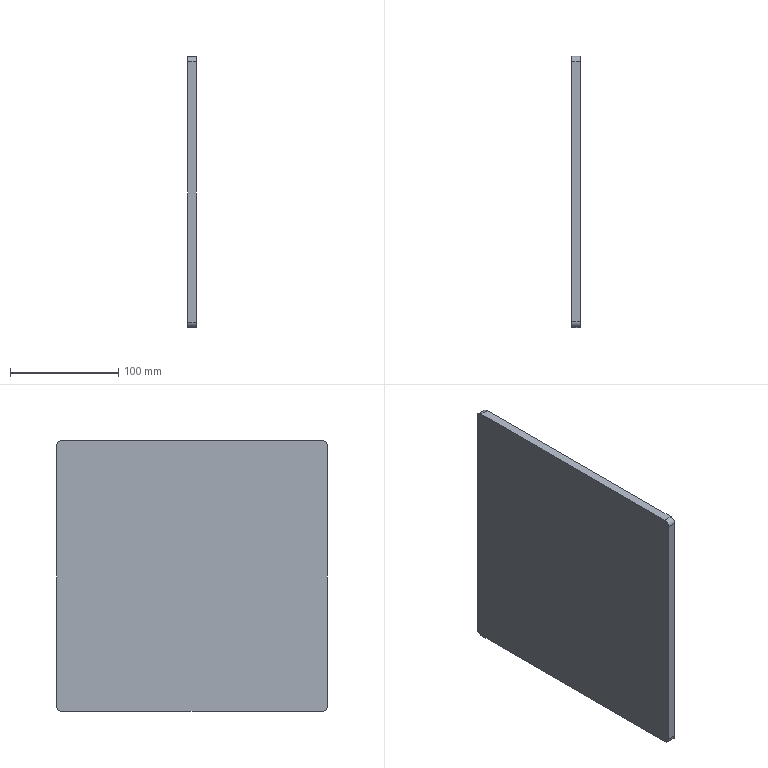Component | SolidWorks | FlipWindow-1 | 1 solid | 10 faces | box 8 x 250 x 250 mm | volume 499828 mm3 | plane 6 | cylinder 4 | commonest cylinder face diameters 10 x4 | material 45
build123d program:
from build123d import *

# Parameters (mm, degrees)
SKETCH1_W           = 250
SKETCH1_H           = 250
BOSS_EXTRUDE1_DEPTH = 8
FILLET1_R           = 5


with BuildPart() as part:
    # Sketch1 → Boss-Extrude1 (new body)
    with BuildSketch(Plane(origin=(0, 0, 0), x_dir=(1, 0, 0), z_dir=(0, 1, 0))):
        Rectangle(SKETCH1_W, SKETCH1_H)
    extrude(amount=BOSS_EXTRUDE1_DEPTH)

    # Fillet1
    fillet1_edges = [part.edges().sort_by_distance(p)[0] for p in [
        (-125, 4, -125),
        (125, 4, -125),
        (125, 4, 125),
        (-125, 4, 125),
    ]]
    fillet(fillet1_edges, radius=FILLET1_R)


solid = part.part

# Placed as in the assembly
solid = solid.moved(Location((-233.359, -177.285, 1075), (0, 0, 90)))
STEP:
#1=COLOUR_RGB('',0.7922,0.8196,0.9333);
#2=FILL_AREA_STYLE_COLOUR('',#1);
#3=FILL_AREA_STYLE('',(#2));
#4=SURFACE_STYLE_FILL_AREA(#3);
#5=SURFACE_SIDE_STYLE('',(#4));
#6=SURFACE_STYLE_USAGE(.BOTH.,#5);
#7=PRESENTATION_STYLE_ASSIGNMENT((#6));
#8=CARTESIAN_POINT('',(-9.187,-11.704,37.402));
#9=VERTEX_POINT('',#8);
#10=CARTESIAN_POINT('',(-9.187,-2.255,37.402));
#11=VERTEX_POINT('',#10);
#12=CARTESIAN_POINT('',(-9.187,-2.058,37.402));
#13=DIRECTION('',(0.,1.,-0.));
#14=VECTOR('',#13,39.37);
#15=LINE('',#12,#14);
#16=EDGE_CURVE('',#9,#11,#15,.T.);
#17=ORIENTED_EDGE('',*,*,#16,.F.);
#18=CARTESIAN_POINT('',(-9.502,-11.704,37.402));
#19=VERTEX_POINT('',#18);
#20=CARTESIAN_POINT('',(-9.187,-11.704,37.402));
#21=DIRECTION('',(-1.,0.,0.));
#22=VECTOR('',#21,39.37);
#23=LINE('',#20,#22);
#24=EDGE_CURVE('',#9,#19,#23,.T.);
#25=ORIENTED_EDGE('',*,*,#24,.T.);
#26=CARTESIAN_POINT('',(-9.502,-2.255,37.402));
#27=VERTEX_POINT('',#26);
#28=CARTESIAN_POINT('',(-9.502,-2.058,37.402));
#29=DIRECTION('',(0.,1.,-0.));
#30=VECTOR('',#29,39.37);
#31=LINE('',#28,#30);
#32=EDGE_CURVE('',#19,#27,#31,.T.);
#33=ORIENTED_EDGE('',*,*,#32,.T.);
#34=CARTESIAN_POINT('',(-9.187,-2.255,37.402));
#35=DIRECTION('',(1.,-0.,0.));
#36=VECTOR('',#35,39.37);
#37=LINE('',#34,#36);
#38=EDGE_CURVE('',#27,#11,#37,.T.);
#39=ORIENTED_EDGE('',*,*,#38,.T.);
#40=EDGE_LOOP('',(#17,#25,#33,#39));
#41=FACE_OUTER_BOUND('',#40,.T.);
#42=CARTESIAN_POINT('',(-9.187,-2.058,37.402));
#43=DIRECTION('',(0.,0.,1.));
#44=DIRECTION('',(-0.,-1.,0.));
#45=AXIS2_PLACEMENT_3D('',#42,#43,#44);
#46=PLANE('',#45);
#47=ADVANCED_FACE('',(#41),#46,.F.);
#48=CARTESIAN_POINT('',(-9.187,-2.058,37.598));
#49=VERTEX_POINT('',#48);
#50=CARTESIAN_POINT('',(-9.187,-2.058,47.047));
#51=VERTEX_POINT('',#50);
#52=CARTESIAN_POINT('',(-9.187,-2.058,47.244));
#53=DIRECTION('',(0.,0.,1.));
#54=VECTOR('',#53,39.37);
#55=LINE('',#52,#54);
#56=EDGE_CURVE('',#49,#51,#55,.T.);
#57=ORIENTED_EDGE('',*,*,#56,.F.);
#58=CARTESIAN_POINT('',(-9.502,-2.058,37.598));
#59=VERTEX_POINT('',#58);
#60=CARTESIAN_POINT('',(-9.187,-2.058,37.598));
#61=DIRECTION('',(-1.,0.,0.));
#62=VECTOR('',#61,39.37);
#63=LINE('',#60,#62);
#64=EDGE_CURVE('',#49,#59,#63,.T.);
#65=ORIENTED_EDGE('',*,*,#64,.T.);
#66=CARTESIAN_POINT('',(-9.502,-2.058,47.047));
#67=VERTEX_POINT('',#66);
#68=CARTESIAN_POINT('',(-9.502,-2.058,47.244));
#69=DIRECTION('',(0.,0.,1.));
#70=VECTOR('',#69,39.37);
#71=LINE('',#68,#70);
#72=EDGE_CURVE('',#59,#67,#71,.T.);
#73=ORIENTED_EDGE('',*,*,#72,.T.);
#74=CARTESIAN_POINT('',(-9.187,-2.058,47.047));
#75=DIRECTION('',(1.,-0.,0.));
#76=VECTOR('',#75,39.37);
#77=LINE('',#74,#76);
#78=EDGE_CURVE('',#67,#51,#77,.T.);
#79=ORIENTED_EDGE('',*,*,#78,.T.);
#80=EDGE_LOOP('',(#57,#65,#73,#79));
#81=FACE_OUTER_BOUND('',#80,.T.);
#82=CARTESIAN_POINT('',(-9.187,-2.058,47.244));
#83=DIRECTION('',(-0.,-1.,0.));
#84=DIRECTION('',(-0.,-0.,-1.));
#85=AXIS2_PLACEMENT_3D('',#82,#83,#84);
#86=PLANE('',#85);
#87=ADVANCED_FACE('',(#81),#86,.F.);
#88=CARTESIAN_POINT('',(-9.502,-2.255,47.244));
#89=VERTEX_POINT('',#88);
#90=CARTESIAN_POINT('',(-9.502,-11.704,47.244));
#91=VERTEX_POINT('',#90);
#92=CARTESIAN_POINT('',(-9.502,-2.058,47.244));
#93=DIRECTION('',(-0.,-1.,0.));
#94=VECTOR('',#93,39.37);
#95=LINE('',#92,#94);
#96=EDGE_CURVE('',#89,#91,#95,.T.);
#97=ORIENTED_EDGE('',*,*,#96,.T.);
#98=CARTESIAN_POINT('',(-9.187,-11.704,47.244));
#99=VERTEX_POINT('',#98);
#100=CARTESIAN_POINT('',(-9.187,-11.704,47.244));
#101=DIRECTION('',(1.,-0.,0.));
#102=VECTOR('',#101,39.37);
#103=LINE('',#100,#102);
#104=EDGE_CURVE('',#91,#99,#103,.T.);
#105=ORIENTED_EDGE('',*,*,#104,.T.);
#106=CARTESIAN_POINT('',(-9.187,-2.255,47.244));
#107=VERTEX_POINT('',#106);
#108=CARTESIAN_POINT('',(-9.187,-2.058,47.244));
#109=DIRECTION('',(-0.,-1.,0.));
#110=VECTOR('',#109,39.37);
#111=LINE('',#108,#110);
#112=EDGE_CURVE('',#107,#99,#111,.T.);
#113=ORIENTED_EDGE('',*,*,#112,.F.);
#114=CARTESIAN_POINT('',(-9.187,-2.255,47.244));
#115=DIRECTION('',(-1.,0.,0.));
#116=VECTOR('',#115,39.37);
#117=LINE('',#114,#116);
#118=EDGE_CURVE('',#107,#89,#117,.T.);
#119=ORIENTED_EDGE('',*,*,#118,.T.);
#120=EDGE_LOOP('',(#97,#105,#113,#119));
#121=FACE_OUTER_BOUND('',#120,.T.);
#122=CARTESIAN_POINT('',(-9.187,-2.058,47.244));
#123=DIRECTION('',(-0.,-0.,-1.));
#124=DIRECTION('',(0.,1.,-0.));
#125=AXIS2_PLACEMENT_3D('',#122,#123,#124);
#126=PLANE('',#125);
#127=ADVANCED_FACE('',(#121),#126,.F.);
#128=CARTESIAN_POINT('',(-9.502,-11.901,47.047));
#129=VERTEX_POINT('',#128);
#130=CARTESIAN_POINT('',(-9.502,-11.901,37.598));
#131=VERTEX_POINT('',#130);
#132=CARTESIAN_POINT('',(-9.502,-11.901,47.244));
#133=DIRECTION('',(-0.,-0.,-1.));
#134=VECTOR('',#133,39.37);
#135=LINE('',#132,#134);
#136=EDGE_CURVE('',#129,#131,#135,.T.);
#137=ORIENTED_EDGE('',*,*,#136,.T.);
#138=CARTESIAN_POINT('',(-9.187,-11.901,37.598));
#139=VERTEX_POINT('',#138);
#140=CARTESIAN_POINT('',(-9.187,-11.901,37.598));
#141=DIRECTION('',(1.,-0.,0.));
#142=VECTOR('',#141,39.37);
#143=LINE('',#140,#142);
#144=EDGE_CURVE('',#131,#139,#143,.T.);
#145=ORIENTED_EDGE('',*,*,#144,.T.);
#146=CARTESIAN_POINT('',(-9.187,-11.901,47.047));
#147=VERTEX_POINT('',#146);
#148=CARTESIAN_POINT('',(-9.187,-11.901,47.244));
#149=DIRECTION('',(-0.,-0.,-1.));
#150=VECTOR('',#149,39.37);
#151=LINE('',#148,#150);
#152=EDGE_CURVE('',#147,#139,#151,.T.);
#153=ORIENTED_EDGE('',*,*,#152,.F.);
#154=CARTESIAN_POINT('',(-9.187,-11.901,47.047));
#155=DIRECTION('',(-1.,0.,0.));
#156=VECTOR('',#155,39.37);
#157=LINE('',#154,#156);
#158=EDGE_CURVE('',#147,#129,#157,.T.);
#159=ORIENTED_EDGE('',*,*,#158,.T.);
#160=EDGE_LOOP('',(#137,#145,#153,#159));
#161=FACE_OUTER_BOUND('',#160,.T.);
#162=CARTESIAN_POINT('',(-9.187,-11.901,47.244));
#163=DIRECTION('',(0.,1.,-0.));
#164=DIRECTION('',(0.,0.,1.));
#165=AXIS2_PLACEMENT_3D('',#162,#163,#164);
#166=PLANE('',#165);
#167=ADVANCED_FACE('',(#161),#166,.F.);
#168=ORIENTED_EDGE('',*,*,#152,.T.);
#169=CARTESIAN_POINT('',(-9.187,-11.704,37.598));
#170=DIRECTION('',(1.,-0.,0.));
#171=DIRECTION('',(0.,1.,0.));
#172=AXIS2_PLACEMENT_3D('',#169,#170,#171);
#173=CIRCLE('',#172,0.1969);
#174=EDGE_CURVE('',#139,#9,#173,.T.);
#175=ORIENTED_EDGE('',*,*,#174,.T.);
#176=ORIENTED_EDGE('',*,*,#16,.T.);
#177=CARTESIAN_POINT('',(-9.187,-2.255,37.598));
#178=DIRECTION('',(1.,-0.,0.));
#179=DIRECTION('',(0.,1.,0.));
#180=AXIS2_PLACEMENT_3D('',#177,#178,#179);
#181=CIRCLE('',#180,0.1969);
#182=EDGE_CURVE('',#11,#49,#181,.T.);
#183=ORIENTED_EDGE('',*,*,#182,.T.);
#184=ORIENTED_EDGE('',*,*,#56,.T.);
#185=CARTESIAN_POINT('',(-9.187,-2.255,47.047));
#186=DIRECTION('',(1.,-0.,0.));
#187=DIRECTION('',(0.,1.,0.));
#188=AXIS2_PLACEMENT_3D('',#185,#186,#187);
#189=CIRCLE('',#188,0.1969);
#190=EDGE_CURVE('',#51,#107,#189,.T.);
#191=ORIENTED_EDGE('',*,*,#190,.T.);
#192=ORIENTED_EDGE('',*,*,#112,.T.);
#193=CARTESIAN_POINT('',(-9.187,-11.704,47.047));
#194=DIRECTION('',(1.,-0.,0.));
#195=DIRECTION('',(0.,1.,0.));
#196=AXIS2_PLACEMENT_3D('',#193,#194,#195);
#197=CIRCLE('',#196,0.1969);
#198=EDGE_CURVE('',#99,#147,#197,.T.);
#199=ORIENTED_EDGE('',*,*,#198,.T.);
#200=EDGE_LOOP('',(#168,#175,#176,#183,#184,#191,#192,#199));
#201=FACE_OUTER_BOUND('',#200,.T.);
#202=CARTESIAN_POINT('',(-9.187,-6.98,42.323));
#203=DIRECTION('',(1.,-0.,0.));
#204=DIRECTION('',(0.,1.,-0.));
#205=AXIS2_PLACEMENT_3D('',#202,#203,#204);
#206=PLANE('',#205);
#207=ADVANCED_FACE('',(#201),#206,.T.);
#208=ORIENTED_EDGE('',*,*,#32,.F.);
#209=CARTESIAN_POINT('',(-9.502,-11.704,37.598));
#210=DIRECTION('',(-1.,0.,0.));
#211=DIRECTION('',(0.,1.,0.));
#212=AXIS2_PLACEMENT_3D('',#209,#210,#211);
#213=CIRCLE('',#212,0.1969);
#214=EDGE_CURVE('',#19,#131,#213,.T.);
#215=ORIENTED_EDGE('',*,*,#214,.T.);
#216=ORIENTED_EDGE('',*,*,#136,.F.);
#217=CARTESIAN_POINT('',(-9.502,-11.704,47.047));
#218=DIRECTION('',(-1.,0.,0.));
#219=DIRECTION('',(0.,1.,0.));
#220=AXIS2_PLACEMENT_3D('',#217,#218,#219);
#221=CIRCLE('',#220,0.1969);
#222=EDGE_CURVE('',#129,#91,#221,.T.);
#223=ORIENTED_EDGE('',*,*,#222,.T.);
#224=ORIENTED_EDGE('',*,*,#96,.F.);
#225=CARTESIAN_POINT('',(-9.502,-2.255,47.047));
#226=DIRECTION('',(-1.,0.,0.));
#227=DIRECTION('',(0.,1.,0.));
#228=AXIS2_PLACEMENT_3D('',#225,#226,#227);
#229=CIRCLE('',#228,0.1969);
#230=EDGE_CURVE('',#89,#67,#229,.T.);
#231=ORIENTED_EDGE('',*,*,#230,.T.);
#232=ORIENTED_EDGE('',*,*,#72,.F.);
#233=CARTESIAN_POINT('',(-9.502,-2.255,37.598));
#234=DIRECTION('',(-1.,0.,0.));
#235=DIRECTION('',(0.,1.,0.));
#236=AXIS2_PLACEMENT_3D('',#233,#234,#235);
#237=CIRCLE('',#236,0.1969);
#238=EDGE_CURVE('',#59,#27,#237,.T.);
#239=ORIENTED_EDGE('',*,*,#238,.T.);
#240=EDGE_LOOP('',(#208,#215,#216,#223,#224,#231,#232,#239));
#241=FACE_OUTER_BOUND('',#240,.T.);
#242=CARTESIAN_POINT('',(-9.502,-6.98,42.323));
#243=DIRECTION('',(1.,-0.,0.));
#244=DIRECTION('',(0.,1.,-0.));
#245=AXIS2_PLACEMENT_3D('',#242,#243,#244);
#246=PLANE('',#245);
#247=ADVANCED_FACE('',(#241),#246,.F.);
#248=ORIENTED_EDGE('',*,*,#174,.F.);
#249=ORIENTED_EDGE('',*,*,#144,.F.);
#250=ORIENTED_EDGE('',*,*,#214,.F.);
#251=ORIENTED_EDGE('',*,*,#24,.F.);
#252=EDGE_LOOP('',(#248,#249,#250,#251));
#253=FACE_OUTER_BOUND('',#252,.T.);
#254=CARTESIAN_POINT('',(-9.187,-11.704,37.598));
#255=DIRECTION('',(-1.,0.,0.));
#256=DIRECTION('',(0.,-1.,0.));
#257=AXIS2_PLACEMENT_3D('',#254,#255,#256);
#258=CYLINDRICAL_SURFACE('',#257,0.1969);
#259=ADVANCED_FACE('',(#253),#258,.T.);
#260=ORIENTED_EDGE('',*,*,#182,.F.);
#261=ORIENTED_EDGE('',*,*,#38,.F.);
#262=ORIENTED_EDGE('',*,*,#238,.F.);
#263=ORIENTED_EDGE('',*,*,#64,.F.);
#264=EDGE_LOOP('',(#260,#261,#262,#263));
#265=FACE_OUTER_BOUND('',#264,.T.);
#266=CARTESIAN_POINT('',(-9.187,-2.255,37.598));
#267=DIRECTION('',(-1.,0.,0.));
#268=DIRECTION('',(0.,-1.,0.));
#269=AXIS2_PLACEMENT_3D('',#266,#267,#268);
#270=CYLINDRICAL_SURFACE('',#269,0.1969);
#271=ADVANCED_FACE('',(#265),#270,.T.);
#272=ORIENTED_EDGE('',*,*,#198,.F.);
#273=ORIENTED_EDGE('',*,*,#104,.F.);
#274=ORIENTED_EDGE('',*,*,#222,.F.);
#275=ORIENTED_EDGE('',*,*,#158,.F.);
#276=EDGE_LOOP('',(#272,#273,#274,#275));
#277=FACE_OUTER_BOUND('',#276,.T.);
#278=CARTESIAN_POINT('',(-9.187,-11.704,47.047));
#279=DIRECTION('',(-1.,0.,0.));
#280=DIRECTION('',(0.,-1.,0.));
#281=AXIS2_PLACEMENT_3D('',#278,#279,#280);
#282=CYLINDRICAL_SURFACE('',#281,0.1969);
#283=ADVANCED_FACE('',(#277),#282,.T.);
#284=ORIENTED_EDGE('',*,*,#190,.F.);
#285=ORIENTED_EDGE('',*,*,#78,.F.);
#286=ORIENTED_EDGE('',*,*,#230,.F.);
#287=ORIENTED_EDGE('',*,*,#118,.F.);
#288=EDGE_LOOP('',(#284,#285,#286,#287));
#289=FACE_OUTER_BOUND('',#288,.T.);
#290=CARTESIAN_POINT('',(-9.187,-2.255,47.047));
#291=DIRECTION('',(-1.,0.,0.));
#292=DIRECTION('',(0.,-1.,0.));
#293=AXIS2_PLACEMENT_3D('',#290,#291,#292);
#294=CYLINDRICAL_SURFACE('',#293,0.1969);
#295=ADVANCED_FACE('',(#289),#294,.T.);
#296=CLOSED_SHELL('',(#47,#87,#127,#167,#207,#247,#259,#271,#283,#295));
#297=MANIFOLD_SOLID_BREP('',#296);
#298=STYLED_ITEM('',(#7),#297);
#299=(LENGTH_UNIT()NAMED_UNIT(*)SI_UNIT($,.METRE.));
#300=LENGTH_MEASURE_WITH_UNIT(LENGTH_MEASURE(0.0254),#299);
#301=DIMENSIONAL_EXPONENTS(1.,0.,0.,0.,0.,0.,0.);
#302=(CONVERSION_BASED_UNIT('',#300)LENGTH_UNIT()NAMED_UNIT(#301));
#303=UNCERTAINTY_MEASURE_WITH_UNIT(LENGTH_MEASURE(0.00001),#302,'','');
#304=(NAMED_UNIT(*)PLANE_ANGLE_UNIT()SI_UNIT($,.RADIAN.));
#305=(NAMED_UNIT(*)SI_UNIT($,.STERADIAN.)SOLID_ANGLE_UNIT());
#306=(GEOMETRIC_REPRESENTATION_CONTEXT(3)GLOBAL_UNCERTAINTY_ASSIGNED_CONTEXT((#303))GLOBAL_UNIT_ASSIGNED_CONTEXT((#302,#304,#305))REPRESENTATION_CONTEXT('',''));
#307=MECHANICAL_DESIGN_GEOMETRIC_PRESENTATION_REPRESENTATION('',(#298),#306);
#308=PRESENTATION_LAYER_ASSIGNMENT('','',(#298));
#309=CARTESIAN_POINT('',(0.,0.,0.));
#310=DIRECTION('',(0.,0.,1.));
#311=DIRECTION('',(1.,0.,0.));
#312=AXIS2_PLACEMENT_3D('',#309,#310,#311);
#313=(LENGTH_UNIT()NAMED_UNIT(*)SI_UNIT($,.METRE.));
#314=LENGTH_MEASURE_WITH_UNIT(LENGTH_MEASURE(0.0254),#313);
#315=DIMENSIONAL_EXPONENTS(1.,0.,0.,0.,0.,0.,0.);
#316=(CONVERSION_BASED_UNIT('',#314)LENGTH_UNIT()NAMED_UNIT(#315));
#317=UNCERTAINTY_MEASURE_WITH_UNIT(LENGTH_MEASURE(0.00001),#316,'','');
#318=(NAMED_UNIT(*)PLANE_ANGLE_UNIT()SI_UNIT($,.RADIAN.));
#319=(NAMED_UNIT(*)SI_UNIT($,.STERADIAN.)SOLID_ANGLE_UNIT());
#320=(GEOMETRIC_REPRESENTATION_CONTEXT(3)GLOBAL_UNCERTAINTY_ASSIGNED_CONTEXT((#317))GLOBAL_UNIT_ASSIGNED_CONTEXT((#316,#318,#319))REPRESENTATION_CONTEXT('',''));
#321=ADVANCED_BREP_SHAPE_REPRESENTATION('',(#297,#312),#320);